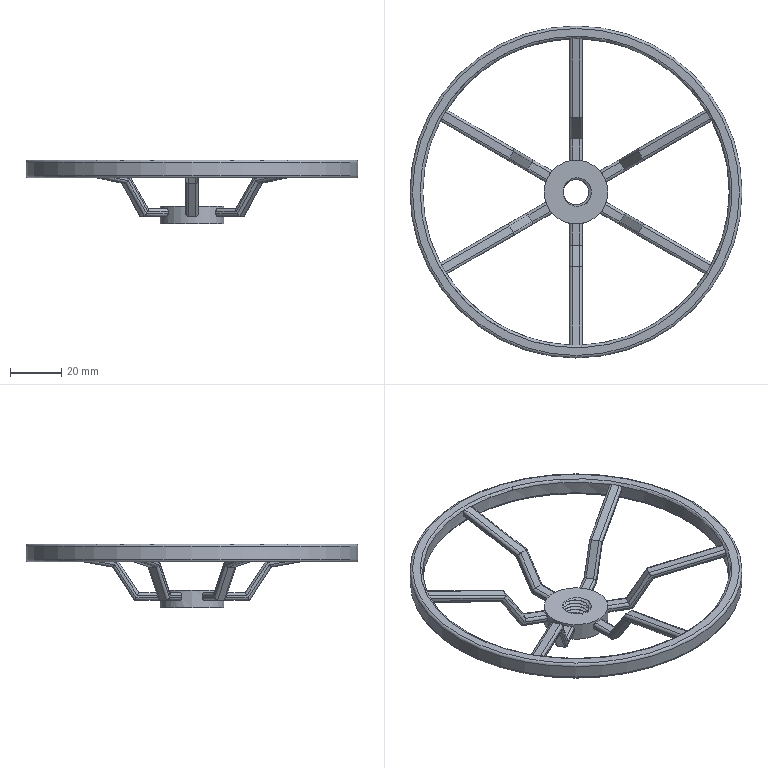Component | NX | HANDWHEEL | 1 solid | 137 faces | volume 20844 mm3 | cylinder 78 | plane 53 | torus 4 | spline 2 | commonest cylinder face diameters 2 x72 120 x2 25 x1 10 x1 130 x1 12 x1